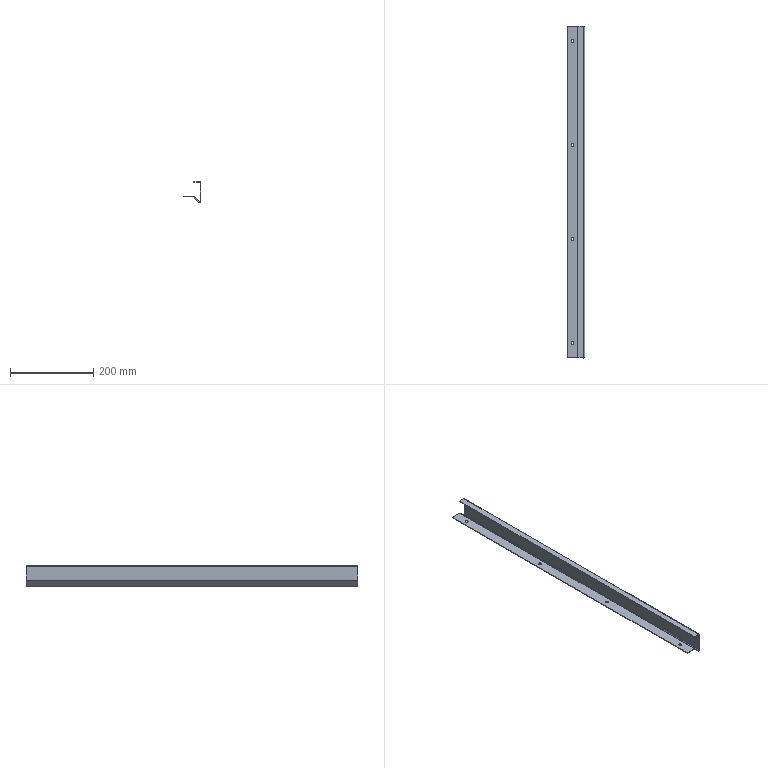Component | SolidWorks | Brow(Item1)-1 | 1 solid | 40 faces | box 42 x 796 x 50 mm | volume 130732 mm3 | plane 24 | cylinder 16 | commonest cylinder face diameters 7 x8 3 x4 6 x4 | material Plain Carbon Steel
STEP:
#1=COLOUR_RGB('',0.7922,0.8196,0.9333);
#2=FILL_AREA_STYLE_COLOUR('',#1);
#3=FILL_AREA_STYLE('',(#2));
#4=SURFACE_STYLE_FILL_AREA(#3);
#5=SURFACE_SIDE_STYLE('',(#4));
#6=SURFACE_STYLE_USAGE(.BOTH.,#5);
#7=PRESENTATION_STYLE_ASSIGNMENT((#6));
#8=CARTESIAN_POINT('',(15.256,14.134,-86.673));
#9=VERTEX_POINT('',#8);
#10=CARTESIAN_POINT('',(15.256,14.409,-86.673));
#11=VERTEX_POINT('',#10);
#12=CARTESIAN_POINT('',(15.256,14.272,-86.673));
#13=DIRECTION('',(0.,-0.,1.));
#14=DIRECTION('',(0.,-1.,0.));
#15=AXIS2_PLACEMENT_3D('',#12,#13,#14);
#16=CIRCLE('',#15,0.1378);
#17=EDGE_CURVE('',#9,#11,#16,.T.);
#18=ORIENTED_EDGE('',*,*,#17,.F.);
#19=CARTESIAN_POINT('',(15.256,14.134,-86.614));
#20=VERTEX_POINT('',#19);
#21=CARTESIAN_POINT('',(15.256,14.134,-87.205));
#22=DIRECTION('',(0.,-0.,1.));
#23=VECTOR('',#22,39.37);
#24=LINE('',#21,#23);
#25=EDGE_CURVE('',#9,#20,#24,.T.);
#26=ORIENTED_EDGE('',*,*,#25,.T.);
#27=CARTESIAN_POINT('',(15.256,14.409,-86.614));
#28=VERTEX_POINT('',#27);
#29=CARTESIAN_POINT('',(15.256,14.272,-86.614));
#30=DIRECTION('',(0.,-0.,1.));
#31=DIRECTION('',(0.,1.,0.));
#32=AXIS2_PLACEMENT_3D('',#29,#30,#31);
#33=CIRCLE('',#32,0.1378);
#34=EDGE_CURVE('',#20,#28,#33,.T.);
#35=ORIENTED_EDGE('',*,*,#34,.T.);
#36=CARTESIAN_POINT('',(15.256,14.409,-87.205));
#37=DIRECTION('',(0.,-0.,1.));
#38=VECTOR('',#37,39.37);
#39=LINE('',#36,#38);
#40=EDGE_CURVE('',#11,#28,#39,.T.);
#41=ORIENTED_EDGE('',*,*,#40,.F.);
#42=EDGE_LOOP('',(#18,#26,#35,#41));
#43=FACE_OUTER_BOUND('',#42,.T.);
#44=CARTESIAN_POINT('',(15.256,14.272,-87.205));
#45=DIRECTION('',(0.,-0.,1.));
#46=DIRECTION('',(0.,1.,0.));
#47=AXIS2_PLACEMENT_3D('',#44,#45,#46);
#48=CYLINDRICAL_SURFACE('',#47,0.1378);
#49=ADVANCED_FACE('',(#43),#48,.F.);
#50=CARTESIAN_POINT('',(15.256,-14.409,-86.673));
#51=VERTEX_POINT('',#50);
#52=CARTESIAN_POINT('',(15.256,-14.134,-86.673));
#53=VERTEX_POINT('',#52);
#54=CARTESIAN_POINT('',(15.256,-14.272,-86.673));
#55=DIRECTION('',(0.,-0.,1.));
#56=DIRECTION('',(0.,-1.,0.));
#57=AXIS2_PLACEMENT_3D('',#54,#55,#56);
#58=CIRCLE('',#57,0.1378);
#59=EDGE_CURVE('',#51,#53,#58,.T.);
#60=ORIENTED_EDGE('',*,*,#59,.F.);
#61=CARTESIAN_POINT('',(15.256,-14.409,-86.614));
#62=VERTEX_POINT('',#61);
#63=CARTESIAN_POINT('',(15.256,-14.409,-87.205));
#64=DIRECTION('',(0.,-0.,1.));
#65=VECTOR('',#64,39.37);
#66=LINE('',#63,#65);
#67=EDGE_CURVE('',#51,#62,#66,.T.);
#68=ORIENTED_EDGE('',*,*,#67,.T.);
#69=CARTESIAN_POINT('',(15.256,-14.134,-86.614));
#70=VERTEX_POINT('',#69);
#71=CARTESIAN_POINT('',(15.256,-14.272,-86.614));
#72=DIRECTION('',(0.,-0.,1.));
#73=DIRECTION('',(0.,1.,0.));
#74=AXIS2_PLACEMENT_3D('',#71,#72,#73);
#75=CIRCLE('',#74,0.1378);
#76=EDGE_CURVE('',#62,#70,#75,.T.);
#77=ORIENTED_EDGE('',*,*,#76,.T.);
#78=CARTESIAN_POINT('',(15.256,-14.134,-87.205));
#79=DIRECTION('',(0.,-0.,1.));
#80=VECTOR('',#79,39.37);
#81=LINE('',#78,#80);
#82=EDGE_CURVE('',#53,#70,#81,.T.);
#83=ORIENTED_EDGE('',*,*,#82,.F.);
#84=EDGE_LOOP('',(#60,#68,#77,#83));
#85=FACE_OUTER_BOUND('',#84,.T.);
#86=CARTESIAN_POINT('',(15.256,-14.272,-87.205));
#87=DIRECTION('',(0.,-0.,1.));
#88=DIRECTION('',(0.,1.,0.));
#89=AXIS2_PLACEMENT_3D('',#86,#87,#88);
#90=CYLINDRICAL_SURFACE('',#89,0.1378);
#91=ADVANCED_FACE('',(#85),#90,.F.);
#92=CARTESIAN_POINT('',(15.256,4.291,-86.673));
#93=VERTEX_POINT('',#92);
#94=CARTESIAN_POINT('',(15.256,4.567,-86.673));
#95=VERTEX_POINT('',#94);
#96=CARTESIAN_POINT('',(15.256,4.429,-86.673));
#97=DIRECTION('',(0.,-0.,1.));
#98=DIRECTION('',(0.,-1.,0.));
#99=AXIS2_PLACEMENT_3D('',#96,#97,#98);
#100=CIRCLE('',#99,0.1378);
#101=EDGE_CURVE('',#93,#95,#100,.T.);
#102=ORIENTED_EDGE('',*,*,#101,.F.);
#103=CARTESIAN_POINT('',(15.256,4.291,-86.614));
#104=VERTEX_POINT('',#103);
#105=CARTESIAN_POINT('',(15.256,4.291,-87.205));
#106=DIRECTION('',(0.,-0.,1.));
#107=VECTOR('',#106,39.37);
#108=LINE('',#105,#107);
#109=EDGE_CURVE('',#93,#104,#108,.T.);
#110=ORIENTED_EDGE('',*,*,#109,.T.);
#111=CARTESIAN_POINT('',(15.256,4.567,-86.614));
#112=VERTEX_POINT('',#111);
#113=CARTESIAN_POINT('',(15.256,4.429,-86.614));
#114=DIRECTION('',(0.,-0.,1.));
#115=DIRECTION('',(0.,-1.,0.));
#116=AXIS2_PLACEMENT_3D('',#113,#114,#115);
#117=CIRCLE('',#116,0.1378);
#118=EDGE_CURVE('',#104,#112,#117,.T.);
#119=ORIENTED_EDGE('',*,*,#118,.T.);
#120=CARTESIAN_POINT('',(15.256,4.567,-87.205));
#121=DIRECTION('',(0.,-0.,1.));
#122=VECTOR('',#121,39.37);
#123=LINE('',#120,#122);
#124=EDGE_CURVE('',#95,#112,#123,.T.);
#125=ORIENTED_EDGE('',*,*,#124,.F.);
#126=EDGE_LOOP('',(#102,#110,#119,#125));
#127=FACE_OUTER_BOUND('',#126,.T.);
#128=CARTESIAN_POINT('',(15.256,4.429,-87.205));
#129=DIRECTION('',(0.,-0.,1.));
#130=DIRECTION('',(0.,1.,0.));
#131=AXIS2_PLACEMENT_3D('',#128,#129,#130);
#132=CYLINDRICAL_SURFACE('',#131,0.1378);
#133=ADVANCED_FACE('',(#127),#132,.F.);
#134=CARTESIAN_POINT('',(15.256,-4.567,-86.673));
#135=VERTEX_POINT('',#134);
#136=CARTESIAN_POINT('',(15.256,-4.291,-86.673));
#137=VERTEX_POINT('',#136);
#138=CARTESIAN_POINT('',(15.256,-4.429,-86.673));
#139=DIRECTION('',(0.,-0.,1.));
#140=DIRECTION('',(0.,-1.,0.));
#141=AXIS2_PLACEMENT_3D('',#138,#139,#140);
#142=CIRCLE('',#141,0.1378);
#143=EDGE_CURVE('',#135,#137,#142,.T.);
#144=ORIENTED_EDGE('',*,*,#143,.F.);
#145=CARTESIAN_POINT('',(15.256,-4.567,-86.614));
#146=VERTEX_POINT('',#145);
#147=CARTESIAN_POINT('',(15.256,-4.567,-87.205));
#148=DIRECTION('',(0.,-0.,1.));
#149=VECTOR('',#148,39.37);
#150=LINE('',#147,#149);
#151=EDGE_CURVE('',#135,#146,#150,.T.);
#152=ORIENTED_EDGE('',*,*,#151,.T.);
#153=CARTESIAN_POINT('',(15.256,-4.291,-86.614));
#154=VERTEX_POINT('',#153);
#155=CARTESIAN_POINT('',(15.256,-4.429,-86.614));
#156=DIRECTION('',(0.,-0.,1.));
#157=DIRECTION('',(0.,1.,0.));
#158=AXIS2_PLACEMENT_3D('',#155,#156,#157);
#159=CIRCLE('',#158,0.1378);
#160=EDGE_CURVE('',#146,#154,#159,.T.);
#161=ORIENTED_EDGE('',*,*,#160,.T.);
#162=CARTESIAN_POINT('',(15.256,-4.291,-87.205));
#163=DIRECTION('',(0.,-0.,1.));
#164=VECTOR('',#163,39.37);
#165=LINE('',#162,#164);
#166=EDGE_CURVE('',#137,#154,#165,.T.);
#167=ORIENTED_EDGE('',*,*,#166,.F.);
#168=EDGE_LOOP('',(#144,#152,#161,#167));
#169=FACE_OUTER_BOUND('',#168,.T.);
#170=CARTESIAN_POINT('',(15.256,-4.429,-87.205));
#171=DIRECTION('',(0.,-0.,1.));
#172=DIRECTION('',(0.,1.,0.));
#173=AXIS2_PLACEMENT_3D('',#170,#171,#172);
#174=CYLINDRICAL_SURFACE('',#173,0.1378);
#175=ADVANCED_FACE('',(#169),#174,.F.);
#176=CARTESIAN_POINT('',(16.299,-15.669,-87.146));
#177=VERTEX_POINT('',#176);
#178=CARTESIAN_POINT('',(16.256,-15.669,-87.127));
#179=VERTEX_POINT('',#178);
#180=CARTESIAN_POINT('',(16.299,-15.669,-87.087));
#181=DIRECTION('',(-0.,1.,0.));
#182=DIRECTION('',(0.,0.,1.));
#183=AXIS2_PLACEMENT_3D('',#180,#181,#182);
#184=CIRCLE('',#183,0.05906);
#185=EDGE_CURVE('',#177,#179,#184,.T.);
#186=ORIENTED_EDGE('',*,*,#185,.F.);
#187=CARTESIAN_POINT('',(16.299,15.669,-87.146));
#188=VERTEX_POINT('',#187);
#189=CARTESIAN_POINT('',(16.299,-15.669,-87.146));
#190=DIRECTION('',(-0.,1.,0.));
#191=VECTOR('',#190,39.37);
#192=LINE('',#189,#191);
#193=EDGE_CURVE('',#177,#188,#192,.T.);
#194=ORIENTED_EDGE('',*,*,#193,.T.);
#195=CARTESIAN_POINT('',(16.256,15.669,-87.127));
#196=VERTEX_POINT('',#195);
#197=CARTESIAN_POINT('',(16.299,15.669,-87.087));
#198=DIRECTION('',(-0.,1.,0.));
#199=DIRECTION('',(0.,0.,1.));
#200=AXIS2_PLACEMENT_3D('',#197,#198,#199);
#201=CIRCLE('',#200,0.05906);
#202=EDGE_CURVE('',#188,#196,#201,.T.);
#203=ORIENTED_EDGE('',*,*,#202,.T.);
#204=CARTESIAN_POINT('',(16.256,-15.669,-87.127));
#205=DIRECTION('',(-0.,1.,0.));
#206=VECTOR('',#205,39.37);
#207=LINE('',#204,#206);
#208=EDGE_CURVE('',#179,#196,#207,.T.);
#209=ORIENTED_EDGE('',*,*,#208,.F.);
#210=EDGE_LOOP('',(#186,#194,#203,#209));
#211=FACE_OUTER_BOUND('',#210,.T.);
#212=CARTESIAN_POINT('',(16.299,-15.669,-87.087));
#213=DIRECTION('',(-0.,1.,0.));
#214=DIRECTION('',(0.,0.,-1.));
#215=AXIS2_PLACEMENT_3D('',#212,#213,#214);
#216=CYLINDRICAL_SURFACE('',#215,0.05906);
#217=ADVANCED_FACE('',(#211),#216,.F.);
#218=CARTESIAN_POINT('',(16.417,-15.669,-87.087));
#219=VERTEX_POINT('',#218);
#220=CARTESIAN_POINT('',(16.299,-15.669,-87.205));
#221=VERTEX_POINT('',#220);
#222=CARTESIAN_POINT('',(16.299,-15.669,-87.087));
#223=DIRECTION('',(-0.,1.,0.));
#224=DIRECTION('',(0.,0.,-1.));
#225=AXIS2_PLACEMENT_3D('',#222,#223,#224);
#226=CIRCLE('',#225,0.1181);
#227=EDGE_CURVE('',#219,#221,#226,.T.);
#228=ORIENTED_EDGE('',*,*,#227,.T.);
#229=CARTESIAN_POINT('',(16.299,15.669,-87.205));
#230=VERTEX_POINT('',#229);
#231=CARTESIAN_POINT('',(16.299,-15.669,-87.205));
#232=DIRECTION('',(-0.,1.,0.));
#233=VECTOR('',#232,39.37);
#234=LINE('',#231,#233);
#235=EDGE_CURVE('',#221,#230,#234,.T.);
#236=ORIENTED_EDGE('',*,*,#235,.T.);
#237=CARTESIAN_POINT('',(16.417,15.669,-87.087));
#238=VERTEX_POINT('',#237);
#239=CARTESIAN_POINT('',(16.299,15.669,-87.087));
#240=DIRECTION('',(-0.,1.,0.));
#241=DIRECTION('',(0.,0.,-1.));
#242=AXIS2_PLACEMENT_3D('',#239,#240,#241);
#243=CIRCLE('',#242,0.1181);
#244=EDGE_CURVE('',#238,#230,#243,.T.);
#245=ORIENTED_EDGE('',*,*,#244,.F.);
#246=CARTESIAN_POINT('',(16.417,-15.669,-87.087));
#247=DIRECTION('',(-0.,1.,0.));
#248=VECTOR('',#247,39.37);
#249=LINE('',#246,#248);
#250=EDGE_CURVE('',#219,#238,#249,.T.);
#251=ORIENTED_EDGE('',*,*,#250,.F.);
#252=EDGE_LOOP('',(#228,#236,#245,#251));
#253=FACE_OUTER_BOUND('',#252,.T.);
#254=CARTESIAN_POINT('',(16.299,-15.669,-87.087));
#255=DIRECTION('',(-0.,1.,0.));
#256=DIRECTION('',(0.,0.,-1.));
#257=AXIS2_PLACEMENT_3D('',#254,#255,#256);
#258=CYLINDRICAL_SURFACE('',#257,0.1181);
#259=ADVANCED_FACE('',(#253),#258,.T.);
#260=CARTESIAN_POINT('',(16.213,-15.669,-87.168));
#261=VERTEX_POINT('',#260);
#262=CARTESIAN_POINT('',(16.213,-15.669,-87.168));
#263=DIRECTION('',(0.7283,0.,0.6853));
#264=VECTOR('',#263,39.37);
#265=LINE('',#262,#264);
#266=EDGE_CURVE('',#261,#179,#265,.T.);
#267=ORIENTED_EDGE('',*,*,#266,.F.);
#268=CARTESIAN_POINT('',(16.299,-15.669,-87.087));
#269=DIRECTION('',(-0.,1.,0.));
#270=DIRECTION('',(0.,0.,-1.));
#271=AXIS2_PLACEMENT_3D('',#268,#269,#270);
#272=CIRCLE('',#271,0.1181);
#273=EDGE_CURVE('',#221,#261,#272,.T.);
#274=ORIENTED_EDGE('',*,*,#273,.F.);
#275=ORIENTED_EDGE('',*,*,#227,.F.);
#276=CARTESIAN_POINT('',(16.358,-15.669,-87.087));
#277=VERTEX_POINT('',#276);
#278=CARTESIAN_POINT('',(16.358,-15.669,-87.087));
#279=DIRECTION('',(1.,0.,-0.));
#280=VECTOR('',#279,39.37);
#281=LINE('',#278,#280);
#282=EDGE_CURVE('',#277,#219,#281,.T.);
#283=ORIENTED_EDGE('',*,*,#282,.F.);
#284=CARTESIAN_POINT('',(16.299,-15.669,-87.087));
#285=DIRECTION('',(-0.,1.,0.));
#286=DIRECTION('',(0.,0.,1.));
#287=AXIS2_PLACEMENT_3D('',#284,#285,#286);
#288=CIRCLE('',#287,0.05906);
#289=EDGE_CURVE('',#277,#177,#288,.T.);
#290=ORIENTED_EDGE('',*,*,#289,.T.);
#291=ORIENTED_EDGE('',*,*,#185,.T.);
#292=EDGE_LOOP('',(#267,#274,#275,#283,#290,#291));
#293=FACE_OUTER_BOUND('',#292,.T.);
#294=CARTESIAN_POINT('',(16.213,-15.669,-87.168));
#295=DIRECTION('',(0.,-1.,-0.));
#296=DIRECTION('',(0.,-0.,1.));
#297=AXIS2_PLACEMENT_3D('',#294,#295,#296);
#298=PLANE('',#297);
#299=ADVANCED_FACE('',(#293),#298,.T.);
#300=CARTESIAN_POINT('',(15.766,-15.669,-86.692));
#301=VERTEX_POINT('',#300);
#302=CARTESIAN_POINT('',(16.213,-15.669,-87.168));
#303=DIRECTION('',(-0.6853,-0.,0.7283));
#304=VECTOR('',#303,39.37);
#305=LINE('',#302,#304);
#306=EDGE_CURVE('',#261,#301,#305,.T.);
#307=ORIENTED_EDGE('',*,*,#306,.F.);
#308=ORIENTED_EDGE('',*,*,#266,.T.);
#309=CARTESIAN_POINT('',(15.809,-15.669,-86.651));
#310=VERTEX_POINT('',#309);
#311=CARTESIAN_POINT('',(16.256,-15.669,-87.127));
#312=DIRECTION('',(-0.6853,-0.,0.7283));
#313=VECTOR('',#312,39.37);
#314=LINE('',#311,#313);
#315=EDGE_CURVE('',#179,#310,#314,.T.);
#316=ORIENTED_EDGE('',*,*,#315,.T.);
#317=CARTESIAN_POINT('',(15.809,-15.669,-86.651));
#318=DIRECTION('',(-0.7283,-0.,-0.6853));
#319=VECTOR('',#318,39.37);
#320=LINE('',#317,#319);
#321=EDGE_CURVE('',#310,#301,#320,.T.);
#322=ORIENTED_EDGE('',*,*,#321,.T.);
#323=EDGE_LOOP('',(#307,#308,#316,#322));
#324=FACE_OUTER_BOUND('',#323,.T.);
#325=CARTESIAN_POINT('',(16.358,-15.669,-87.087));
#326=DIRECTION('',(0.,-1.,-0.));
#327=DIRECTION('',(0.,-0.,1.));
#328=AXIS2_PLACEMENT_3D('',#325,#326,#327);
#329=PLANE('',#328);
#330=ADVANCED_FACE('',(#324),#329,.T.);
#331=CARTESIAN_POINT('',(16.358,15.669,-87.087));
#332=VERTEX_POINT('',#331);
#333=CARTESIAN_POINT('',(16.417,15.669,-87.087));
#334=DIRECTION('',(-1.,-0.,0.));
#335=VECTOR('',#334,39.37);
#336=LINE('',#333,#335);
#337=EDGE_CURVE('',#238,#332,#336,.T.);
#338=ORIENTED_EDGE('',*,*,#337,.F.);
#339=ORIENTED_EDGE('',*,*,#244,.T.);
#340=CARTESIAN_POINT('',(16.213,15.669,-87.168));
#341=VERTEX_POINT('',#340);
#342=CARTESIAN_POINT('',(16.299,15.669,-87.087));
#343=DIRECTION('',(-0.,1.,0.));
#344=DIRECTION('',(0.,0.,-1.));
#345=AXIS2_PLACEMENT_3D('',#342,#343,#344);
#346=CIRCLE('',#345,0.1181);
#347=EDGE_CURVE('',#230,#341,#346,.T.);
#348=ORIENTED_EDGE('',*,*,#347,.T.);
#349=CARTESIAN_POINT('',(16.256,15.669,-87.127));
#350=DIRECTION('',(-0.7283,-0.,-0.6853));
#351=VECTOR('',#350,39.37);
#352=LINE('',#349,#351);
#353=EDGE_CURVE('',#196,#341,#352,.T.);
#354=ORIENTED_EDGE('',*,*,#353,.F.);
#355=ORIENTED_EDGE('',*,*,#202,.F.);
#356=CARTESIAN_POINT('',(16.299,15.669,-87.087));
#357=DIRECTION('',(-0.,1.,0.));
#358=DIRECTION('',(0.,0.,1.));
#359=AXIS2_PLACEMENT_3D('',#356,#357,#358);
#360=CIRCLE('',#359,0.05906);
#361=EDGE_CURVE('',#332,#188,#360,.T.);
#362=ORIENTED_EDGE('',*,*,#361,.F.);
#363=EDGE_LOOP('',(#338,#339,#348,#354,#355,#362));
#364=FACE_OUTER_BOUND('',#363,.T.);
#365=CARTESIAN_POINT('',(16.417,15.669,-87.087));
#366=DIRECTION('',(-0.,1.,0.));
#367=DIRECTION('',(-0.,0.,-1.));
#368=AXIS2_PLACEMENT_3D('',#365,#366,#367);
#369=PLANE('',#368);
#370=ADVANCED_FACE('',(#364),#369,.T.);
#371=CARTESIAN_POINT('',(16.417,15.669,-85.354));
#372=VERTEX_POINT('',#371);
#373=CARTESIAN_POINT('',(16.417,15.669,-85.236));
#374=DIRECTION('',(-0.,0.,-1.));
#375=VECTOR('',#374,39.37);
#376=LINE('',#373,#375);
#377=EDGE_CURVE('',#372,#238,#376,.T.);
#378=ORIENTED_EDGE('',*,*,#377,.T.);
#379=ORIENTED_EDGE('',*,*,#337,.T.);
#380=CARTESIAN_POINT('',(16.358,15.669,-85.354));
#381=VERTEX_POINT('',#380);
#382=CARTESIAN_POINT('',(16.358,15.669,-85.236));
#383=DIRECTION('',(-0.,0.,-1.));
#384=VECTOR('',#383,39.37);
#385=LINE('',#382,#384);
#386=EDGE_CURVE('',#381,#332,#385,.T.);
#387=ORIENTED_EDGE('',*,*,#386,.F.);
#388=CARTESIAN_POINT('',(16.358,15.669,-85.354));
#389=DIRECTION('',(1.,0.,-0.));
#390=VECTOR('',#389,39.37);
#391=LINE('',#388,#390);
#392=EDGE_CURVE('',#381,#372,#391,.T.);
#393=ORIENTED_EDGE('',*,*,#392,.T.);
#394=EDGE_LOOP('',(#378,#379,#387,#393));
#395=FACE_OUTER_BOUND('',#394,.T.);
#396=CARTESIAN_POINT('',(16.256,15.669,-87.127));
#397=DIRECTION('',(-0.,1.,0.));
#398=DIRECTION('',(-0.,0.,-1.));
#399=AXIS2_PLACEMENT_3D('',#396,#397,#398);
#400=PLANE('',#399);
#401=ADVANCED_FACE('',(#395),#400,.T.);
#402=CARTESIAN_POINT('',(16.417,-15.669,-85.354));
#403=VERTEX_POINT('',#402);
#404=CARTESIAN_POINT('',(16.358,-15.669,-85.354));
#405=VERTEX_POINT('',#404);
#406=CARTESIAN_POINT('',(16.417,-15.669,-85.354));
#407=DIRECTION('',(-1.,-0.,0.));
#408=VECTOR('',#407,39.37);
#409=LINE('',#406,#408);
#410=EDGE_CURVE('',#403,#405,#409,.T.);
#411=ORIENTED_EDGE('',*,*,#410,.F.);
#412=CARTESIAN_POINT('',(16.299,-15.669,-85.236));
#413=VERTEX_POINT('',#412);
#414=CARTESIAN_POINT('',(16.299,-15.669,-85.354));
#415=DIRECTION('',(-0.,1.,0.));
#416=DIRECTION('',(0.,0.,1.));
#417=AXIS2_PLACEMENT_3D('',#414,#415,#416);
#418=CIRCLE('',#417,0.1181);
#419=EDGE_CURVE('',#413,#403,#418,.T.);
#420=ORIENTED_EDGE('',*,*,#419,.F.);
#421=CARTESIAN_POINT('',(16.299,-15.669,-85.295));
#422=VERTEX_POINT('',#421);
#423=CARTESIAN_POINT('',(16.299,-15.669,-85.295));
#424=DIRECTION('',(0.,-0.,1.));
#425=VECTOR('',#424,39.37);
#426=LINE('',#423,#425);
#427=EDGE_CURVE('',#422,#413,#426,.T.);
#428=ORIENTED_EDGE('',*,*,#427,.F.);
#429=CARTESIAN_POINT('',(16.299,-15.669,-85.354));
#430=DIRECTION('',(-0.,1.,0.));
#431=DIRECTION('',(0.,0.,1.));
#432=AXIS2_PLACEMENT_3D('',#429,#430,#431);
#433=CIRCLE('',#432,0.05906);
#434=EDGE_CURVE('',#422,#405,#433,.T.);
#435=ORIENTED_EDGE('',*,*,#434,.T.);
#436=EDGE_LOOP('',(#411,#420,#428,#435));
#437=FACE_OUTER_BOUND('',#436,.T.);
#438=CARTESIAN_POINT('',(16.417,-15.669,-85.354));
#439=DIRECTION('',(0.,-1.,-0.));
#440=DIRECTION('',(0.,-0.,1.));
#441=AXIS2_PLACEMENT_3D('',#438,#439,#440);
#442=PLANE('',#441);
#443=ADVANCED_FACE('',(#437),#442,.T.);
#444=CARTESIAN_POINT('',(16.417,-15.669,-85.236));
#445=DIRECTION('',(-0.,0.,-1.));
#446=VECTOR('',#445,39.37);
#447=LINE('',#444,#446);
#448=EDGE_CURVE('',#403,#219,#447,.T.);
#449=ORIENTED_EDGE('',*,*,#448,.F.);
#450=ORIENTED_EDGE('',*,*,#410,.T.);
#451=CARTESIAN_POINT('',(16.358,-15.669,-85.236));
#452=DIRECTION('',(-0.,0.,-1.));
#453=VECTOR('',#452,39.37);
#454=LINE('',#451,#453);
#455=EDGE_CURVE('',#405,#277,#454,.T.);
#456=ORIENTED_EDGE('',*,*,#455,.T.);
#457=ORIENTED_EDGE('',*,*,#282,.T.);
#458=EDGE_LOOP('',(#449,#450,#456,#457));
#459=FACE_OUTER_BOUND('',#458,.T.);
#460=CARTESIAN_POINT('',(16.299,-15.669,-85.295));
#461=DIRECTION('',(0.,-1.,-0.));
#462=DIRECTION('',(0.,-0.,1.));
#463=AXIS2_PLACEMENT_3D('',#460,#461,#462);
#464=PLANE('',#463);
#465=ADVANCED_FACE('',(#459),#464,.T.);
#466=CARTESIAN_POINT('',(16.299,15.669,-85.236));
#467=VERTEX_POINT('',#466);
#468=CARTESIAN_POINT('',(16.299,15.669,-85.295));
#469=VERTEX_POINT('',#468);
#470=CARTESIAN_POINT('',(16.299,15.669,-85.236));
#471=DIRECTION('',(-0.,0.,-1.));
#472=VECTOR('',#471,39.37);
#473=LINE('',#470,#472);
#474=EDGE_CURVE('',#467,#469,#473,.T.);
#475=ORIENTED_EDGE('',*,*,#474,.F.);
#476=CARTESIAN_POINT('',(16.299,15.669,-85.354));
#477=DIRECTION('',(-0.,1.,0.));
#478=DIRECTION('',(0.,0.,1.));
#479=AXIS2_PLACEMENT_3D('',#476,#477,#478);
#480=CIRCLE('',#479,0.1181);
#481=EDGE_CURVE('',#467,#372,#480,.T.);
#482=ORIENTED_EDGE('',*,*,#481,.T.);
#483=ORIENTED_EDGE('',*,*,#392,.F.);
#484=CARTESIAN_POINT('',(16.299,15.669,-85.354));
#485=DIRECTION('',(-0.,1.,0.));
#486=DIRECTION('',(0.,0.,1.));
#487=AXIS2_PLACEMENT_3D('',#484,#485,#486);
#488=CIRCLE('',#487,0.05906);
#489=EDGE_CURVE('',#469,#381,#488,.T.);
#490=ORIENTED_EDGE('',*,*,#489,.F.);
#491=EDGE_LOOP('',(#475,#482,#483,#490));
#492=FACE_OUTER_BOUND('',#491,.T.);
#493=CARTESIAN_POINT('',(16.299,15.669,-85.236));
#494=DIRECTION('',(-0.,1.,0.));
#495=DIRECTION('',(-0.,0.,-1.));
#496=AXIS2_PLACEMENT_3D('',#493,#494,#495);
#497=PLANE('',#496);
#498=ADVANCED_FACE('',(#492),#497,.T.);
#499=CARTESIAN_POINT('',(15.748,15.669,-85.236));
#500=VERTEX_POINT('',#499);
#501=CARTESIAN_POINT('',(15.748,15.669,-85.236));
#502=DIRECTION('',(1.,0.,-0.));
#503=VECTOR('',#502,39.37);
#504=LINE('',#501,#503);
#505=EDGE_CURVE('',#500,#467,#504,.T.);
#506=ORIENTED_EDGE('',*,*,#505,.T.);
#507=ORIENTED_EDGE('',*,*,#474,.T.);
#508=CARTESIAN_POINT('',(15.748,15.669,-85.295));
#509=VERTEX_POINT('',#508);
#510=CARTESIAN_POINT('',(15.748,15.669,-85.295));
#511=DIRECTION('',(1.,0.,-0.));
#512=VECTOR('',#511,39.37);
#513=LINE('',#510,#512);
#514=EDGE_CURVE('',#509,#469,#513,.T.);
#515=ORIENTED_EDGE('',*,*,#514,.F.);
#516=CARTESIAN_POINT('',(15.748,15.669,-85.295));
#517=DIRECTION('',(0.,-0.,1.));
#518=VECTOR('',#517,39.37);
#519=LINE('',#516,#518);
#520=EDGE_CURVE('',#509,#500,#519,.T.);
#521=ORIENTED_EDGE('',*,*,#520,.T.);
#522=EDGE_LOOP('',(#506,#507,#515,#521));
#523=FACE_OUTER_BOUND('',#522,.T.);
#524=CARTESIAN_POINT('',(16.358,15.669,-85.354));
#525=DIRECTION('',(-0.,1.,0.));
#526=DIRECTION('',(-0.,0.,-1.));
#527=AXIS2_PLACEMENT_3D('',#524,#525,#526);
#528=PLANE('',#527);
#529=ADVANCED_FACE('',(#523),#528,.T.);
#530=CARTESIAN_POINT('',(15.723,-15.669,-86.673));
#531=VERTEX_POINT('',#530);
#532=CARTESIAN_POINT('',(15.723,-15.669,-86.614));
#533=VERTEX_POINT('',#532);
#534=CARTESIAN_POINT('',(15.723,-15.669,-86.673));
#535=DIRECTION('',(0.,-0.,1.));
#536=VECTOR('',#535,39.37);
#537=LINE('',#534,#536);
#538=EDGE_CURVE('',#531,#533,#537,.T.);
#539=ORIENTED_EDGE('',*,*,#538,.F.);
#540=CARTESIAN_POINT('',(15.723,-15.669,-86.732));
#541=DIRECTION('',(0.,-1.,-0.));
#542=DIRECTION('',(0.,0.,-1.));
#543=AXIS2_PLACEMENT_3D('',#540,#541,#542);
#544=CIRCLE('',#543,0.05906);
#545=EDGE_CURVE('',#301,#531,#544,.T.);
#546=ORIENTED_EDGE('',*,*,#545,.F.);
#547=ORIENTED_EDGE('',*,*,#321,.F.);
#548=CARTESIAN_POINT('',(15.723,-15.669,-86.732));
#549=DIRECTION('',(0.,-1.,-0.));
#550=DIRECTION('',(0.,0.,1.));
#551=AXIS2_PLACEMENT_3D('',#548,#549,#550);
#552=CIRCLE('',#551,0.1181);
#553=EDGE_CURVE('',#310,#533,#552,.T.);
#554=ORIENTED_EDGE('',*,*,#553,.T.);
#555=EDGE_LOOP('',(#539,#546,#547,#554));
#556=FACE_OUTER_BOUND('',#555,.T.);
#557=CARTESIAN_POINT('',(15.723,-15.669,-86.673));
#558=DIRECTION('',(0.,-1.,-0.));
#559=DIRECTION('',(0.,-0.,1.));
#560=AXIS2_PLACEMENT_3D('',#557,#558,#559);
#561=PLANE('',#560);
#562=ADVANCED_FACE('',(#556),#561,.T.);
#563=CARTESIAN_POINT('',(14.764,-15.669,-86.673));
#564=VERTEX_POINT('',#563);
#565=CARTESIAN_POINT('',(15.748,-15.669,-86.673));
#566=DIRECTION('',(-1.,-0.,0.));
#567=VECTOR('',#566,39.37);
#568=LINE('',#565,#567);
#569=EDGE_CURVE('',#531,#564,#568,.T.);
#570=ORIENTED_EDGE('',*,*,#569,.F.);
#571=ORIENTED_EDGE('',*,*,#538,.T.);
#572=CARTESIAN_POINT('',(14.764,-15.669,-86.614));
#573=VERTEX_POINT('',#572);
#574=CARTESIAN_POINT('',(15.748,-15.669,-86.614));
#575=DIRECTION('',(-1.,-0.,0.));
#576=VECTOR('',#575,39.37);
#577=LINE('',#574,#576);
#578=EDGE_CURVE('',#533,#573,#577,.T.);
#579=ORIENTED_EDGE('',*,*,#578,.T.);
#580=CARTESIAN_POINT('',(14.764,-15.669,-86.673));
#581=DIRECTION('',(0.,-0.,1.));
#582=VECTOR('',#581,39.37);
#583=LINE('',#580,#582);
#584=EDGE_CURVE('',#564,#573,#583,.T.);
#585=ORIENTED_EDGE('',*,*,#584,.F.);
#586=EDGE_LOOP('',(#570,#571,#579,#585));
#587=FACE_OUTER_BOUND('',#586,.T.);
#588=CARTESIAN_POINT('',(15.809,-15.669,-86.651));
#589=DIRECTION('',(0.,-1.,-0.));
#590=DIRECTION('',(0.,-0.,1.));
#591=AXIS2_PLACEMENT_3D('',#588,#589,#590);
#592=PLANE('',#591);
#593=ADVANCED_FACE('',(#587),#592,.T.);
#594=CARTESIAN_POINT('',(15.766,15.669,-86.692));
#595=VERTEX_POINT('',#594);
#596=CARTESIAN_POINT('',(15.809,15.669,-86.651));
#597=VERTEX_POINT('',#596);
#598=CARTESIAN_POINT('',(15.766,15.669,-86.692));
#599=DIRECTION('',(0.7283,0.,0.6853));
#600=VECTOR('',#599,39.37);
#601=LINE('',#598,#600);
#602=EDGE_CURVE('',#595,#597,#601,.T.);
#603=ORIENTED_EDGE('',*,*,#602,.F.);
#604=CARTESIAN_POINT('',(15.723,15.669,-86.673));
#605=VERTEX_POINT('',#604);
#606=CARTESIAN_POINT('',(15.723,15.669,-86.732));
#607=DIRECTION('',(0.,-1.,-0.));
#608=DIRECTION('',(0.,0.,-1.));
#609=AXIS2_PLACEMENT_3D('',#606,#607,#608);
#610=CIRCLE('',#609,0.05906);
#611=EDGE_CURVE('',#595,#605,#610,.T.);
#612=ORIENTED_EDGE('',*,*,#611,.T.);
#613=CARTESIAN_POINT('',(15.723,15.669,-86.614));
#614=VERTEX_POINT('',#613);
#615=CARTESIAN_POINT('',(15.723,15.669,-86.614));
#616=DIRECTION('',(-0.,0.,-1.));
#617=VECTOR('',#616,39.37);
#618=LINE('',#615,#617);
#619=EDGE_CURVE('',#614,#605,#618,.T.);
#620=ORIENTED_EDGE('',*,*,#619,.F.);
#621=CARTESIAN_POINT('',(15.723,15.669,-86.732));
#622=DIRECTION('',(0.,-1.,-0.));
#623=DIRECTION('',(0.,0.,1.));
#624=AXIS2_PLACEMENT_3D('',#621,#622,#623);
#625=CIRCLE('',#624,0.1181);
#626=EDGE_CURVE('',#597,#614,#625,.T.);
#627=ORIENTED_EDGE('',*,*,#626,.F.);
#628=EDGE_LOOP('',(#603,#612,#620,#627));
#629=FACE_OUTER_BOUND('',#628,.T.);
#630=CARTESIAN_POINT('',(15.766,15.669,-86.692));
#631=DIRECTION('',(-0.,1.,0.));
#632=DIRECTION('',(-0.,0.,-1.));
#633=AXIS2_PLACEMENT_3D('',#630,#631,#632);
#634=PLANE('',#633);
#635=ADVANCED_FACE('',(#629),#634,.T.);
#636=CARTESIAN_POINT('',(16.213,15.669,-87.168));
#637=DIRECTION('',(-0.6853,-0.,0.7283));
#638=VECTOR('',#637,39.37);
#639=LINE('',#636,#638);
#640=EDGE_CURVE('',#341,#595,#639,.T.);
#641=ORIENTED_EDGE('',*,*,#640,.T.);
#642=ORIENTED_EDGE('',*,*,#602,.T.);
#643=CARTESIAN_POINT('',(16.256,15.669,-87.127));
#644=DIRECTION('',(-0.6853,-0.,0.7283));
#645=VECTOR('',#644,39.37);
#646=LINE('',#643,#645);
#647=EDGE_CURVE('',#196,#597,#646,.T.);
#648=ORIENTED_EDGE('',*,*,#647,.F.);
#649=ORIENTED_EDGE('',*,*,#353,.T.);
#650=EDGE_LOOP('',(#641,#642,#648,#649));
#651=FACE_OUTER_BOUND('',#650,.T.);
#652=CARTESIAN_POINT('',(15.723,15.669,-86.614));
#653=DIRECTION('',(-0.,1.,0.));
#654=DIRECTION('',(-0.,0.,-1.));
#655=AXIS2_PLACEMENT_3D('',#652,#653,#654);
#656=PLANE('',#655);
#657=ADVANCED_FACE('',(#651),#656,.T.);
#658=CARTESIAN_POINT('',(15.256,14.272,-86.614));
#659=DIRECTION('',(0.,-0.,1.));
#660=DIRECTION('',(0.,1.,0.));
#661=AXIS2_PLACEMENT_3D('',#658,#659,#660);
#662=CIRCLE('',#661,0.1378);
#663=EDGE_CURVE('',#28,#20,#662,.T.);
#664=ORIENTED_EDGE('',*,*,#663,.F.);
#665=ORIENTED_EDGE('',*,*,#34,.F.);
#666=EDGE_LOOP('',(#664,#665));
#667=FACE_BOUND('',#666,.T.);
#668=CARTESIAN_POINT('',(15.256,-14.272,-86.614));
#669=DIRECTION('',(0.,-0.,1.));
#670=DIRECTION('',(0.,1.,0.));
#671=AXIS2_PLACEMENT_3D('',#668,#669,#670);
#672=CIRCLE('',#671,0.1378);
#673=EDGE_CURVE('',#70,#62,#672,.T.);
#674=ORIENTED_EDGE('',*,*,#673,.F.);
#675=ORIENTED_EDGE('',*,*,#76,.F.);
#676=EDGE_LOOP('',(#674,#675));
#677=FACE_BOUND('',#676,.T.);
#678=CARTESIAN_POINT('',(15.256,4.429,-86.614));
#679=DIRECTION('',(0.,-0.,1.));
#680=DIRECTION('',(0.,-1.,0.));
#681=AXIS2_PLACEMENT_3D('',#678,#679,#680);
#682=CIRCLE('',#681,0.1378);
#683=EDGE_CURVE('',#112,#104,#682,.T.);
#684=ORIENTED_EDGE('',*,*,#683,.F.);
#685=ORIENTED_EDGE('',*,*,#118,.F.);
#686=EDGE_LOOP('',(#684,#685));
#687=FACE_BOUND('',#686,.T.);
#688=CARTESIAN_POINT('',(15.256,-4.429,-86.614));
#689=DIRECTION('',(0.,-0.,1.));
#690=DIRECTION('',(0.,1.,0.));
#691=AXIS2_PLACEMENT_3D('',#688,#689,#690);
#692=CIRCLE('',#691,0.1378);
#693=EDGE_CURVE('',#154,#146,#692,.T.);
#694=ORIENTED_EDGE('',*,*,#693,.F.);
#695=ORIENTED_EDGE('',*,*,#160,.F.);
#696=EDGE_LOOP('',(#694,#695));
#697=FACE_BOUND('',#696,.T.);
#698=CARTESIAN_POINT('',(14.764,15.669,-86.614));
#699=VERTEX_POINT('',#698);
#700=CARTESIAN_POINT('',(15.748,15.669,-86.614));
#701=DIRECTION('',(-1.,-0.,0.));
#702=VECTOR('',#701,39.37);
#703=LINE('',#700,#702);
#704=EDGE_CURVE('',#614,#699,#703,.T.);
#705=ORIENTED_EDGE('',*,*,#704,.T.);
#706=CARTESIAN_POINT('',(14.764,-15.669,-86.614));
#707=DIRECTION('',(-0.,1.,0.));
#708=VECTOR('',#707,39.37);
#709=LINE('',#706,#708);
#710=EDGE_CURVE('',#573,#699,#709,.T.);
#711=ORIENTED_EDGE('',*,*,#710,.F.);
#712=ORIENTED_EDGE('',*,*,#578,.F.);
#713=CARTESIAN_POINT('',(15.723,-15.669,-86.614));
#714=DIRECTION('',(-0.,1.,0.));
#715=VECTOR('',#714,39.37);
#716=LINE('',#713,#715);
#717=EDGE_CURVE('',#533,#614,#716,.T.);
#718=ORIENTED_EDGE('',*,*,#717,.T.);
#719=EDGE_LOOP('',(#705,#711,#712,#718));
#720=FACE_OUTER_BOUND('',#719,.T.);
#721=CARTESIAN_POINT('',(15.748,-15.669,-86.614));
#722=DIRECTION('',(-0.,0.,-1.));
#723=DIRECTION('',(0.,-1.,-0.));
#724=AXIS2_PLACEMENT_3D('',#721,#722,#723);
#725=PLANE('',#724);
#726=ADVANCED_FACE('',(#667,#677,#687,#697,#720),#725,.F.);
#727=CARTESIAN_POINT('',(14.764,15.669,-86.673));
#728=VERTEX_POINT('',#727);
#729=CARTESIAN_POINT('',(14.764,15.669,-86.673));
#730=DIRECTION('',(0.,-0.,1.));
#731=VECTOR('',#730,39.37);
#732=LINE('',#729,#731);
#733=EDGE_CURVE('',#728,#699,#732,.T.);
#734=ORIENTED_EDGE('',*,*,#733,.F.);
#735=CARTESIAN_POINT('',(14.764,-15.669,-86.673));
#736=DIRECTION('',(-0.,1.,0.));
#737=VECTOR('',#736,39.37);
#738=LINE('',#735,#737);
#739=EDGE_CURVE('',#564,#728,#738,.T.);
#740=ORIENTED_EDGE('',*,*,#739,.F.);
#741=ORIENTED_EDGE('',*,*,#584,.T.);
#742=ORIENTED_EDGE('',*,*,#710,.T.);
#743=EDGE_LOOP('',(#734,#740,#741,#742));
#744=FACE_OUTER_BOUND('',#743,.T.);
#745=CARTESIAN_POINT('',(14.764,-15.669,-86.673));
#746=DIRECTION('',(-1.,-0.,0.));
#747=DIRECTION('',(0.,-1.,-0.));
#748=AXIS2_PLACEMENT_3D('',#745,#746,#747);
#749=PLANE('',#748);
#750=ADVANCED_FACE('',(#744),#749,.T.);
#751=CARTESIAN_POINT('',(15.256,14.272,-86.673));
#752=DIRECTION('',(0.,-0.,1.));
#753=DIRECTION('',(0.,-1.,0.));
#754=AXIS2_PLACEMENT_3D('',#751,#752,#753);
#755=CIRCLE('',#754,0.1378);
#756=EDGE_CURVE('',#11,#9,#755,.T.);
#757=ORIENTED_EDGE('',*,*,#756,.T.);
#758=ORIENTED_EDGE('',*,*,#17,.T.);
#759=EDGE_LOOP('',(#757,#758));
#760=FACE_BOUND('',#759,.T.);
#761=CARTESIAN_POINT('',(15.256,-14.272,-86.673));
#762=DIRECTION('',(0.,-0.,1.));
#763=DIRECTION('',(0.,-1.,0.));
#764=AXIS2_PLACEMENT_3D('',#761,#762,#763);
#765=CIRCLE('',#764,0.1378);
#766=EDGE_CURVE('',#53,#51,#765,.T.);
#767=ORIENTED_EDGE('',*,*,#766,.T.);
#768=ORIENTED_EDGE('',*,*,#59,.T.);
#769=EDGE_LOOP('',(#767,#768));
#770=FACE_BOUND('',#769,.T.);
#771=CARTESIAN_POINT('',(15.256,4.429,-86.673));
#772=DIRECTION('',(0.,-0.,1.));
#773=DIRECTION('',(0.,-1.,0.));
#774=AXIS2_PLACEMENT_3D('',#771,#772,#773);
#775=CIRCLE('',#774,0.1378);
#776=EDGE_CURVE('',#95,#93,#775,.T.);
#777=ORIENTED_EDGE('',*,*,#776,.T.);
#778=ORIENTED_EDGE('',*,*,#101,.T.);
#779=EDGE_LOOP('',(#777,#778));
#780=FACE_BOUND('',#779,.T.);
#781=CARTESIAN_POINT('',(15.256,-4.429,-86.673));
#782=DIRECTION('',(0.,-0.,1.));
#783=DIRECTION('',(-0.,-1.,0.));
#784=AXIS2_PLACEMENT_3D('',#781,#782,#783);
#785=CIRCLE('',#784,0.1378);
#786=EDGE_CURVE('',#137,#135,#785,.T.);
#787=ORIENTED_EDGE('',*,*,#786,.T.);
#788=ORIENTED_EDGE('',*,*,#143,.T.);
#789=EDGE_LOOP('',(#787,#788));
#790=FACE_BOUND('',#789,.T.);
#791=CARTESIAN_POINT('',(15.748,15.669,-86.673));
#792=DIRECTION('',(-1.,-0.,0.));
#793=VECTOR('',#792,39.37);
#794=LINE('',#791,#793);
#795=EDGE_CURVE('',#605,#728,#794,.T.);
#796=ORIENTED_EDGE('',*,*,#795,.F.);
#797=CARTESIAN_POINT('',(15.723,-15.669,-86.673));
#798=DIRECTION('',(-0.,1.,0.));
#799=VECTOR('',#798,39.37);
#800=LINE('',#797,#799);
#801=EDGE_CURVE('',#531,#605,#800,.T.);
#802=ORIENTED_EDGE('',*,*,#801,.F.);
#803=ORIENTED_EDGE('',*,*,#569,.T.);
#804=ORIENTED_EDGE('',*,*,#739,.T.);
#805=EDGE_LOOP('',(#796,#802,#803,#804));
#806=FACE_OUTER_BOUND('',#805,.T.);
#807=CARTESIAN_POINT('',(15.748,-15.669,-86.673));
#808=DIRECTION('',(-0.,0.,-1.));
#809=DIRECTION('',(0.,-1.,-0.));
#810=AXIS2_PLACEMENT_3D('',#807,#808,#809);
#811=PLANE('',#810);
#812=ADVANCED_FACE('',(#760,#770,#780,#790,#806),#811,.T.);
#813=ORIENTED_EDGE('',*,*,#611,.F.);
#814=CARTESIAN_POINT('',(15.766,-15.669,-86.692));
#815=DIRECTION('',(-0.,1.,0.));
#816=VECTOR('',#815,39.37);
#817=LINE('',#814,#816);
#818=EDGE_CURVE('',#301,#595,#817,.T.);
#819=ORIENTED_EDGE('',*,*,#818,.F.);
#820=ORIENTED_EDGE('',*,*,#545,.T.);
#821=ORIENTED_EDGE('',*,*,#801,.T.);
#822=EDGE_LOOP('',(#813,#819,#820,#821));
#823=FACE_OUTER_BOUND('',#822,.T.);
#824=CARTESIAN_POINT('',(15.723,-15.669,-86.732));
#825=DIRECTION('',(-0.,1.,0.));
#826=DIRECTION('',(0.,0.,-1.));
#827=AXIS2_PLACEMENT_3D('',#824,#825,#826);
#828=CYLINDRICAL_SURFACE('',#827,0.05906);
#829=ADVANCED_FACE('',(#823),#828,.F.);
#830=ORIENTED_EDGE('',*,*,#640,.F.);
#831=CARTESIAN_POINT('',(16.213,-15.669,-87.168));
#832=DIRECTION('',(-0.,1.,0.));
#833=VECTOR('',#832,39.37);
#834=LINE('',#831,#833);
#835=EDGE_CURVE('',#261,#341,#834,.T.);
#836=ORIENTED_EDGE('',*,*,#835,.F.);
#837=ORIENTED_EDGE('',*,*,#306,.T.);
#838=ORIENTED_EDGE('',*,*,#818,.T.);
#839=EDGE_LOOP('',(#830,#836,#837,#838));
#840=FACE_OUTER_BOUND('',#839,.T.);
#841=CARTESIAN_POINT('',(16.213,-15.669,-87.168));
#842=DIRECTION('',(-0.7283,-0.,-0.6853));
#843=DIRECTION('',(0.6853,0.,-0.7283));
#844=AXIS2_PLACEMENT_3D('',#841,#842,#843);
#845=PLANE('',#844);
#846=ADVANCED_FACE('',(#840),#845,.T.);
#847=ORIENTED_EDGE('',*,*,#235,.F.);
#848=ORIENTED_EDGE('',*,*,#273,.T.);
#849=ORIENTED_EDGE('',*,*,#835,.T.);
#850=ORIENTED_EDGE('',*,*,#347,.F.);
#851=EDGE_LOOP('',(#847,#848,#849,#850));
#852=FACE_OUTER_BOUND('',#851,.T.);
#853=CARTESIAN_POINT('',(16.299,-15.669,-87.087));
#854=DIRECTION('',(-0.,1.,0.));
#855=DIRECTION('',(0.,0.,-1.));
#856=AXIS2_PLACEMENT_3D('',#853,#854,#855);
#857=CYLINDRICAL_SURFACE('',#856,0.1181);
#858=ADVANCED_FACE('',(#852),#857,.T.);
#859=ORIENTED_EDGE('',*,*,#377,.F.);
#860=CARTESIAN_POINT('',(16.417,-15.669,-85.354));
#861=DIRECTION('',(-0.,1.,0.));
#862=VECTOR('',#861,39.37);
#863=LINE('',#860,#862);
#864=EDGE_CURVE('',#403,#372,#863,.T.);
#865=ORIENTED_EDGE('',*,*,#864,.F.);
#866=ORIENTED_EDGE('',*,*,#448,.T.);
#867=ORIENTED_EDGE('',*,*,#250,.T.);
#868=EDGE_LOOP('',(#859,#865,#866,#867));
#869=FACE_OUTER_BOUND('',#868,.T.);
#870=CARTESIAN_POINT('',(16.417,-15.669,-85.236));
#871=DIRECTION('',(1.,0.,-0.));
#872=DIRECTION('',(0.,-0.,1.));
#873=AXIS2_PLACEMENT_3D('',#870,#871,#872);
#874=PLANE('',#873);
#875=ADVANCED_FACE('',(#869),#874,.T.);
#876=ORIENTED_EDGE('',*,*,#481,.F.);
#877=CARTESIAN_POINT('',(16.299,-15.669,-85.236));
#878=DIRECTION('',(-0.,1.,0.));
#879=VECTOR('',#878,39.37);
#880=LINE('',#877,#879);
#881=EDGE_CURVE('',#413,#467,#880,.T.);
#882=ORIENTED_EDGE('',*,*,#881,.F.);
#883=ORIENTED_EDGE('',*,*,#419,.T.);
#884=ORIENTED_EDGE('',*,*,#864,.T.);
#885=EDGE_LOOP('',(#876,#882,#883,#884));
#886=FACE_OUTER_BOUND('',#885,.T.);
#887=CARTESIAN_POINT('',(16.299,-15.669,-85.354));
#888=DIRECTION('',(-0.,1.,0.));
#889=DIRECTION('',(0.,0.,-1.));
#890=AXIS2_PLACEMENT_3D('',#887,#888,#889);
#891=CYLINDRICAL_SURFACE('',#890,0.1181);
#892=ADVANCED_FACE('',(#886),#891,.T.);
#893=ORIENTED_EDGE('',*,*,#505,.F.);
#894=CARTESIAN_POINT('',(15.748,-15.669,-85.236));
#895=VERTEX_POINT('',#894);
#896=CARTESIAN_POINT('',(15.748,-15.669,-85.236));
#897=DIRECTION('',(-0.,1.,0.));
#898=VECTOR('',#897,39.37);
#899=LINE('',#896,#898);
#900=EDGE_CURVE('',#895,#500,#899,.T.);
#901=ORIENTED_EDGE('',*,*,#900,.F.);
#902=CARTESIAN_POINT('',(15.748,-15.669,-85.236));
#903=DIRECTION('',(1.,0.,-0.));
#904=VECTOR('',#903,39.37);
#905=LINE('',#902,#904);
#906=EDGE_CURVE('',#895,#413,#905,.T.);
#907=ORIENTED_EDGE('',*,*,#906,.T.);
#908=ORIENTED_EDGE('',*,*,#881,.T.);
#909=EDGE_LOOP('',(#893,#901,#907,#908));
#910=FACE_OUTER_BOUND('',#909,.T.);
#911=CARTESIAN_POINT('',(15.748,-15.669,-85.236));
#912=DIRECTION('',(0.,-0.,1.));
#913=DIRECTION('',(-1.,-0.,0.));
#914=AXIS2_PLACEMENT_3D('',#911,#912,#913);
#915=PLANE('',#914);
#916=ADVANCED_FACE('',(#910),#915,.T.);
#917=ORIENTED_EDGE('',*,*,#520,.F.);
#918=CARTESIAN_POINT('',(15.748,-15.669,-85.295));
#919=VERTEX_POINT('',#918);
#920=CARTESIAN_POINT('',(15.748,-15.669,-85.295));
#921=DIRECTION('',(-0.,1.,0.));
#922=VECTOR('',#921,39.37);
#923=LINE('',#920,#922);
#924=EDGE_CURVE('',#919,#509,#923,.T.);
#925=ORIENTED_EDGE('',*,*,#924,.F.);
#926=CARTESIAN_POINT('',(15.748,-15.669,-85.295));
#927=DIRECTION('',(0.,-0.,1.));
#928=VECTOR('',#927,39.37);
#929=LINE('',#926,#928);
#930=EDGE_CURVE('',#919,#895,#929,.T.);
#931=ORIENTED_EDGE('',*,*,#930,.T.);
#932=ORIENTED_EDGE('',*,*,#900,.T.);
#933=EDGE_LOOP('',(#917,#925,#931,#932));
#934=FACE_OUTER_BOUND('',#933,.T.);
#935=CARTESIAN_POINT('',(15.748,-15.669,-85.295));
#936=DIRECTION('',(-1.,-0.,0.));
#937=DIRECTION('',(-0.,0.,-1.));
#938=AXIS2_PLACEMENT_3D('',#935,#936,#937);
#939=PLANE('',#938);
#940=ADVANCED_FACE('',(#934),#939,.T.);
#941=ORIENTED_EDGE('',*,*,#514,.T.);
#942=CARTESIAN_POINT('',(16.299,-15.669,-85.295));
#943=DIRECTION('',(-0.,1.,0.));
#944=VECTOR('',#943,39.37);
#945=LINE('',#942,#944);
#946=EDGE_CURVE('',#422,#469,#945,.T.);
#947=ORIENTED_EDGE('',*,*,#946,.F.);
#948=CARTESIAN_POINT('',(15.748,-15.669,-85.295));
#949=DIRECTION('',(1.,0.,-0.));
#950=VECTOR('',#949,39.37);
#951=LINE('',#948,#950);
#952=EDGE_CURVE('',#919,#422,#951,.T.);
#953=ORIENTED_EDGE('',*,*,#952,.F.);
#954=ORIENTED_EDGE('',*,*,#924,.T.);
#955=EDGE_LOOP('',(#941,#947,#953,#954));
#956=FACE_OUTER_BOUND('',#955,.T.);
#957=CARTESIAN_POINT('',(15.748,-15.669,-85.295));
#958=DIRECTION('',(0.,-0.,1.));
#959=DIRECTION('',(-1.,-0.,0.));
#960=AXIS2_PLACEMENT_3D('',#957,#958,#959);
#961=PLANE('',#960);
#962=ADVANCED_FACE('',(#956),#961,.F.);
#963=ORIENTED_EDGE('',*,*,#489,.T.);
#964=CARTESIAN_POINT('',(16.358,-15.669,-85.354));
#965=DIRECTION('',(-0.,1.,0.));
#966=VECTOR('',#965,39.37);
#967=LINE('',#964,#966);
#968=EDGE_CURVE('',#405,#381,#967,.T.);
#969=ORIENTED_EDGE('',*,*,#968,.F.);
#970=ORIENTED_EDGE('',*,*,#434,.F.);
#971=ORIENTED_EDGE('',*,*,#946,.T.);
#972=EDGE_LOOP('',(#963,#969,#970,#971));
#973=FACE_OUTER_BOUND('',#972,.T.);
#974=CARTESIAN_POINT('',(16.299,-15.669,-85.354));
#975=DIRECTION('',(-0.,1.,0.));
#976=DIRECTION('',(0.,0.,-1.));
#977=AXIS2_PLACEMENT_3D('',#974,#975,#976);
#978=CYLINDRICAL_SURFACE('',#977,0.05906);
#979=ADVANCED_FACE('',(#973),#978,.F.);
#980=ORIENTED_EDGE('',*,*,#386,.T.);
#981=CARTESIAN_POINT('',(16.358,-15.669,-87.087));
#982=DIRECTION('',(-0.,1.,0.));
#983=VECTOR('',#982,39.37);
#984=LINE('',#981,#983);
#985=EDGE_CURVE('',#277,#332,#984,.T.);
#986=ORIENTED_EDGE('',*,*,#985,.F.);
#987=ORIENTED_EDGE('',*,*,#455,.F.);
#988=ORIENTED_EDGE('',*,*,#968,.T.);
#989=EDGE_LOOP('',(#980,#986,#987,#988));
#990=FACE_OUTER_BOUND('',#989,.T.);
#991=CARTESIAN_POINT('',(16.358,-15.669,-85.236));
#992=DIRECTION('',(1.,0.,-0.));
#993=DIRECTION('',(0.,-0.,1.));
#994=AXIS2_PLACEMENT_3D('',#991,#992,#993);
#995=PLANE('',#994);
#996=ADVANCED_FACE('',(#990),#995,.F.);
#997=ORIENTED_EDGE('',*,*,#193,.F.);
#998=ORIENTED_EDGE('',*,*,#289,.F.);
#999=ORIENTED_EDGE('',*,*,#985,.T.);
#1000=ORIENTED_EDGE('',*,*,#361,.T.);
#1001=EDGE_LOOP('',(#997,#998,#999,#1000));
#1002=FACE_OUTER_BOUND('',#1001,.T.);
#1003=CARTESIAN_POINT('',(16.299,-15.669,-87.087));
#1004=DIRECTION('',(-0.,1.,0.));
#1005=DIRECTION('',(0.,0.,-1.));
#1006=AXIS2_PLACEMENT_3D('',#1003,#1004,#1005);
#1007=CYLINDRICAL_SURFACE('',#1006,0.05906);
#1008=ADVANCED_FACE('',(#1002),#1007,.F.);
#1009=ORIENTED_EDGE('',*,*,#647,.T.);
#1010=CARTESIAN_POINT('',(15.809,-15.669,-86.651));
#1011=DIRECTION('',(-0.,1.,0.));
#1012=VECTOR('',#1011,39.37);
#1013=LINE('',#1010,#1012);
#1014=EDGE_CURVE('',#310,#597,#1013,.T.);
#1015=ORIENTED_EDGE('',*,*,#1014,.F.);
#1016=ORIENTED_EDGE('',*,*,#315,.F.);
#1017=ORIENTED_EDGE('',*,*,#208,.T.);
#1018=EDGE_LOOP('',(#1009,#1015,#1016,#1017));
#1019=FACE_OUTER_BOUND('',#1018,.T.);
#1020=CARTESIAN_POINT('',(16.256,-15.669,-87.127));
#1021=DIRECTION('',(-0.7283,-0.,-0.6853));
#1022=DIRECTION('',(0.6853,0.,-0.7283));
#1023=AXIS2_PLACEMENT_3D('',#1020,#1021,#1022);
#1024=PLANE('',#1023);
#1025=ADVANCED_FACE('',(#1019),#1024,.F.);
#1026=ORIENTED_EDGE('',*,*,#626,.T.);
#1027=ORIENTED_EDGE('',*,*,#717,.F.);
#1028=ORIENTED_EDGE('',*,*,#553,.F.);
#1029=ORIENTED_EDGE('',*,*,#1014,.T.);
#1030=EDGE_LOOP('',(#1026,#1027,#1028,#1029));
#1031=FACE_OUTER_BOUND('',#1030,.T.);
#1032=CARTESIAN_POINT('',(15.723,-15.669,-86.732));
#1033=DIRECTION('',(-0.,1.,0.));
#1034=DIRECTION('',(0.,0.,-1.));
#1035=AXIS2_PLACEMENT_3D('',#1032,#1033,#1034);
#1036=CYLINDRICAL_SURFACE('',#1035,0.1181);
#1037=ADVANCED_FACE('',(#1031),#1036,.T.);
#1038=ORIENTED_EDGE('',*,*,#952,.T.);
#1039=ORIENTED_EDGE('',*,*,#427,.T.);
#1040=ORIENTED_EDGE('',*,*,#906,.F.);
#1041=ORIENTED_EDGE('',*,*,#930,.F.);
#1042=EDGE_LOOP('',(#1038,#1039,#1040,#1041));
#1043=FACE_OUTER_BOUND('',#1042,.T.);
#1044=CARTESIAN_POINT('',(15.723,-15.669,-86.732));
#1045=DIRECTION('',(-0.,1.,0.));
#1046=DIRECTION('',(-0.,0.,-1.));
#1047=AXIS2_PLACEMENT_3D('',#1044,#1045,#1046);
#1048=PLANE('',#1047);
#1049=ADVANCED_FACE('',(#1043),#1048,.F.);
#1050=ORIENTED_EDGE('',*,*,#704,.F.);
#1051=ORIENTED_EDGE('',*,*,#619,.T.);
#1052=ORIENTED_EDGE('',*,*,#795,.T.);
#1053=ORIENTED_EDGE('',*,*,#733,.T.);
#1054=EDGE_LOOP('',(#1050,#1051,#1052,#1053));
#1055=FACE_OUTER_BOUND('',#1054,.T.);
#1056=CARTESIAN_POINT('',(15.723,15.669,-86.732));
#1057=DIRECTION('',(-0.,1.,0.));
#1058=DIRECTION('',(-0.,0.,-1.));
#1059=AXIS2_PLACEMENT_3D('',#1056,#1057,#1058);
#1060=PLANE('',#1059);
#1061=ADVANCED_FACE('',(#1055),#1060,.T.);
#1062=ORIENTED_EDGE('',*,*,#151,.F.);
#1063=ORIENTED_EDGE('',*,*,#786,.F.);
#1064=ORIENTED_EDGE('',*,*,#166,.T.);
#1065=ORIENTED_EDGE('',*,*,#693,.T.);
#1066=EDGE_LOOP('',(#1062,#1063,#1064,#1065));
#1067=FACE_OUTER_BOUND('',#1066,.T.);
#1068=CARTESIAN_POINT('',(15.256,-4.429,-87.205));
#1069=DIRECTION('',(0.,-0.,1.));
#1070=DIRECTION('',(0.,1.,0.));
#1071=AXIS2_PLACEMENT_3D('',#1068,#1069,#1070);
#1072=CYLINDRICAL_SURFACE('',#1071,0.1378);
#1073=ADVANCED_FACE('',(#1067),#1072,.F.);
#1074=ORIENTED_EDGE('',*,*,#109,.F.);
#1075=ORIENTED_EDGE('',*,*,#776,.F.);
#1076=ORIENTED_EDGE('',*,*,#124,.T.);
#1077=ORIENTED_EDGE('',*,*,#683,.T.);
#1078=EDGE_LOOP('',(#1074,#1075,#1076,#1077));
#1079=FACE_OUTER_BOUND('',#1078,.T.);
#1080=CARTESIAN_POINT('',(15.256,4.429,-87.205));
#1081=DIRECTION('',(0.,-0.,1.));
#1082=DIRECTION('',(0.,1.,0.));
#1083=AXIS2_PLACEMENT_3D('',#1080,#1081,#1082);
#1084=CYLINDRICAL_SURFACE('',#1083,0.1378);
#1085=ADVANCED_FACE('',(#1079),#1084,.F.);
#1086=ORIENTED_EDGE('',*,*,#67,.F.);
#1087=ORIENTED_EDGE('',*,*,#766,.F.);
#1088=ORIENTED_EDGE('',*,*,#82,.T.);
#1089=ORIENTED_EDGE('',*,*,#673,.T.);
#1090=EDGE_LOOP('',(#1086,#1087,#1088,#1089));
#1091=FACE_OUTER_BOUND('',#1090,.T.);
#1092=CARTESIAN_POINT('',(15.256,-14.272,-87.205));
#1093=DIRECTION('',(0.,-0.,1.));
#1094=DIRECTION('',(0.,1.,0.));
#1095=AXIS2_PLACEMENT_3D('',#1092,#1093,#1094);
#1096=CYLINDRICAL_SURFACE('',#1095,0.1378);
#1097=ADVANCED_FACE('',(#1091),#1096,.F.);
#1098=ORIENTED_EDGE('',*,*,#25,.F.);
#1099=ORIENTED_EDGE('',*,*,#756,.F.);
#1100=ORIENTED_EDGE('',*,*,#40,.T.);
#1101=ORIENTED_EDGE('',*,*,#663,.T.);
#1102=EDGE_LOOP('',(#1098,#1099,#1100,#1101));
#1103=FACE_OUTER_BOUND('',#1102,.T.);
#1104=CARTESIAN_POINT('',(15.256,14.272,-87.205));
#1105=DIRECTION('',(0.,-0.,1.));
#1106=DIRECTION('',(0.,1.,0.));
#1107=AXIS2_PLACEMENT_3D('',#1104,#1105,#1106);
#1108=CYLINDRICAL_SURFACE('',#1107,0.1378);
#1109=ADVANCED_FACE('',(#1103),#1108,.F.);
#1110=CLOSED_SHELL('',(#49,#91,#133,#175,#217,#259,#299,#330,#370,#401,#443,#465,#498,#529,#562,#593,#635,#657,#726,#750,#812,#829,#846,#858,#875,#892,#916,#940,#962,#979,#996,#1008,#1025,#1037,#1049,#1061,#1073,#1085,#1097,#1109));
#1111=MANIFOLD_SOLID_BREP('',#1110);
#1112=STYLED_ITEM('',(#7),#1111);
#1113=PRESENTATION_LAYER_ASSIGNMENT('','',(#1112));
#1114=CARTESIAN_POINT('',(0.,0.,0.));
#1115=DIRECTION('',(0.,0.,1.));
#1116=DIRECTION('',(1.,0.,0.));
#1117=AXIS2_PLACEMENT_3D('',#1114,#1115,#1116);
#1118=(LENGTH_UNIT()NAMED_UNIT(*)SI_UNIT($,.METRE.));
#1119=LENGTH_MEASURE_WITH_UNIT(LENGTH_MEASURE(0.0254),#1118);
#1120=DIMENSIONAL_EXPONENTS(1.,0.,0.,0.,0.,0.,0.);
#1121=(CONVERSION_BASED_UNIT('',#1119)LENGTH_UNIT()NAMED_UNIT(#1120));
#1122=UNCERTAINTY_MEASURE_WITH_UNIT(LENGTH_MEASURE(0.00001),#1121,'','');
#1123=(NAMED_UNIT(*)PLANE_ANGLE_UNIT()SI_UNIT($,.RADIAN.));
#1124=(NAMED_UNIT(*)SI_UNIT($,.STERADIAN.)SOLID_ANGLE_UNIT());
#1125=(GEOMETRIC_REPRESENTATION_CONTEXT(3)GLOBAL_UNCERTAINTY_ASSIGNED_CONTEXT((#1122))GLOBAL_UNIT_ASSIGNED_CONTEXT((#1121,#1123,#1124))REPRESENTATION_CONTEXT('',''));
#1126=ADVANCED_BREP_SHAPE_REPRESENTATION('',(#1111,#1117),#1125);
#1127=(LENGTH_UNIT()NAMED_UNIT(*)SI_UNIT($,.METRE.));
#1128=LENGTH_MEASURE_WITH_UNIT(LENGTH_MEASURE(0.0254),#1127);
#1129=DIMENSIONAL_EXPONENTS(1.,0.,0.,0.,0.,0.,0.);
#1130=(CONVERSION_BASED_UNIT('',#1128)LENGTH_UNIT()NAMED_UNIT(#1129));
#1131=UNCERTAINTY_MEASURE_WITH_UNIT(LENGTH_MEASURE(0.00001),#1130,'','');
#1132=(NAMED_UNIT(*)PLANE_ANGLE_UNIT()SI_UNIT($,.RADIAN.));
#1133=(NAMED_UNIT(*)SI_UNIT($,.STERADIAN.)SOLID_ANGLE_UNIT());
#1134=(GEOMETRIC_REPRESENTATION_CONTEXT(3)GLOBAL_UNCERTAINTY_ASSIGNED_CONTEXT((#1131))GLOBAL_UNIT_ASSIGNED_CONTEXT((#1130,#1132,#1133))REPRESENTATION_CONTEXT('',''));
#1135=MECHANICAL_DESIGN_GEOMETRIC_PRESENTATION_REPRESENTATION('',(#1112),#1134);